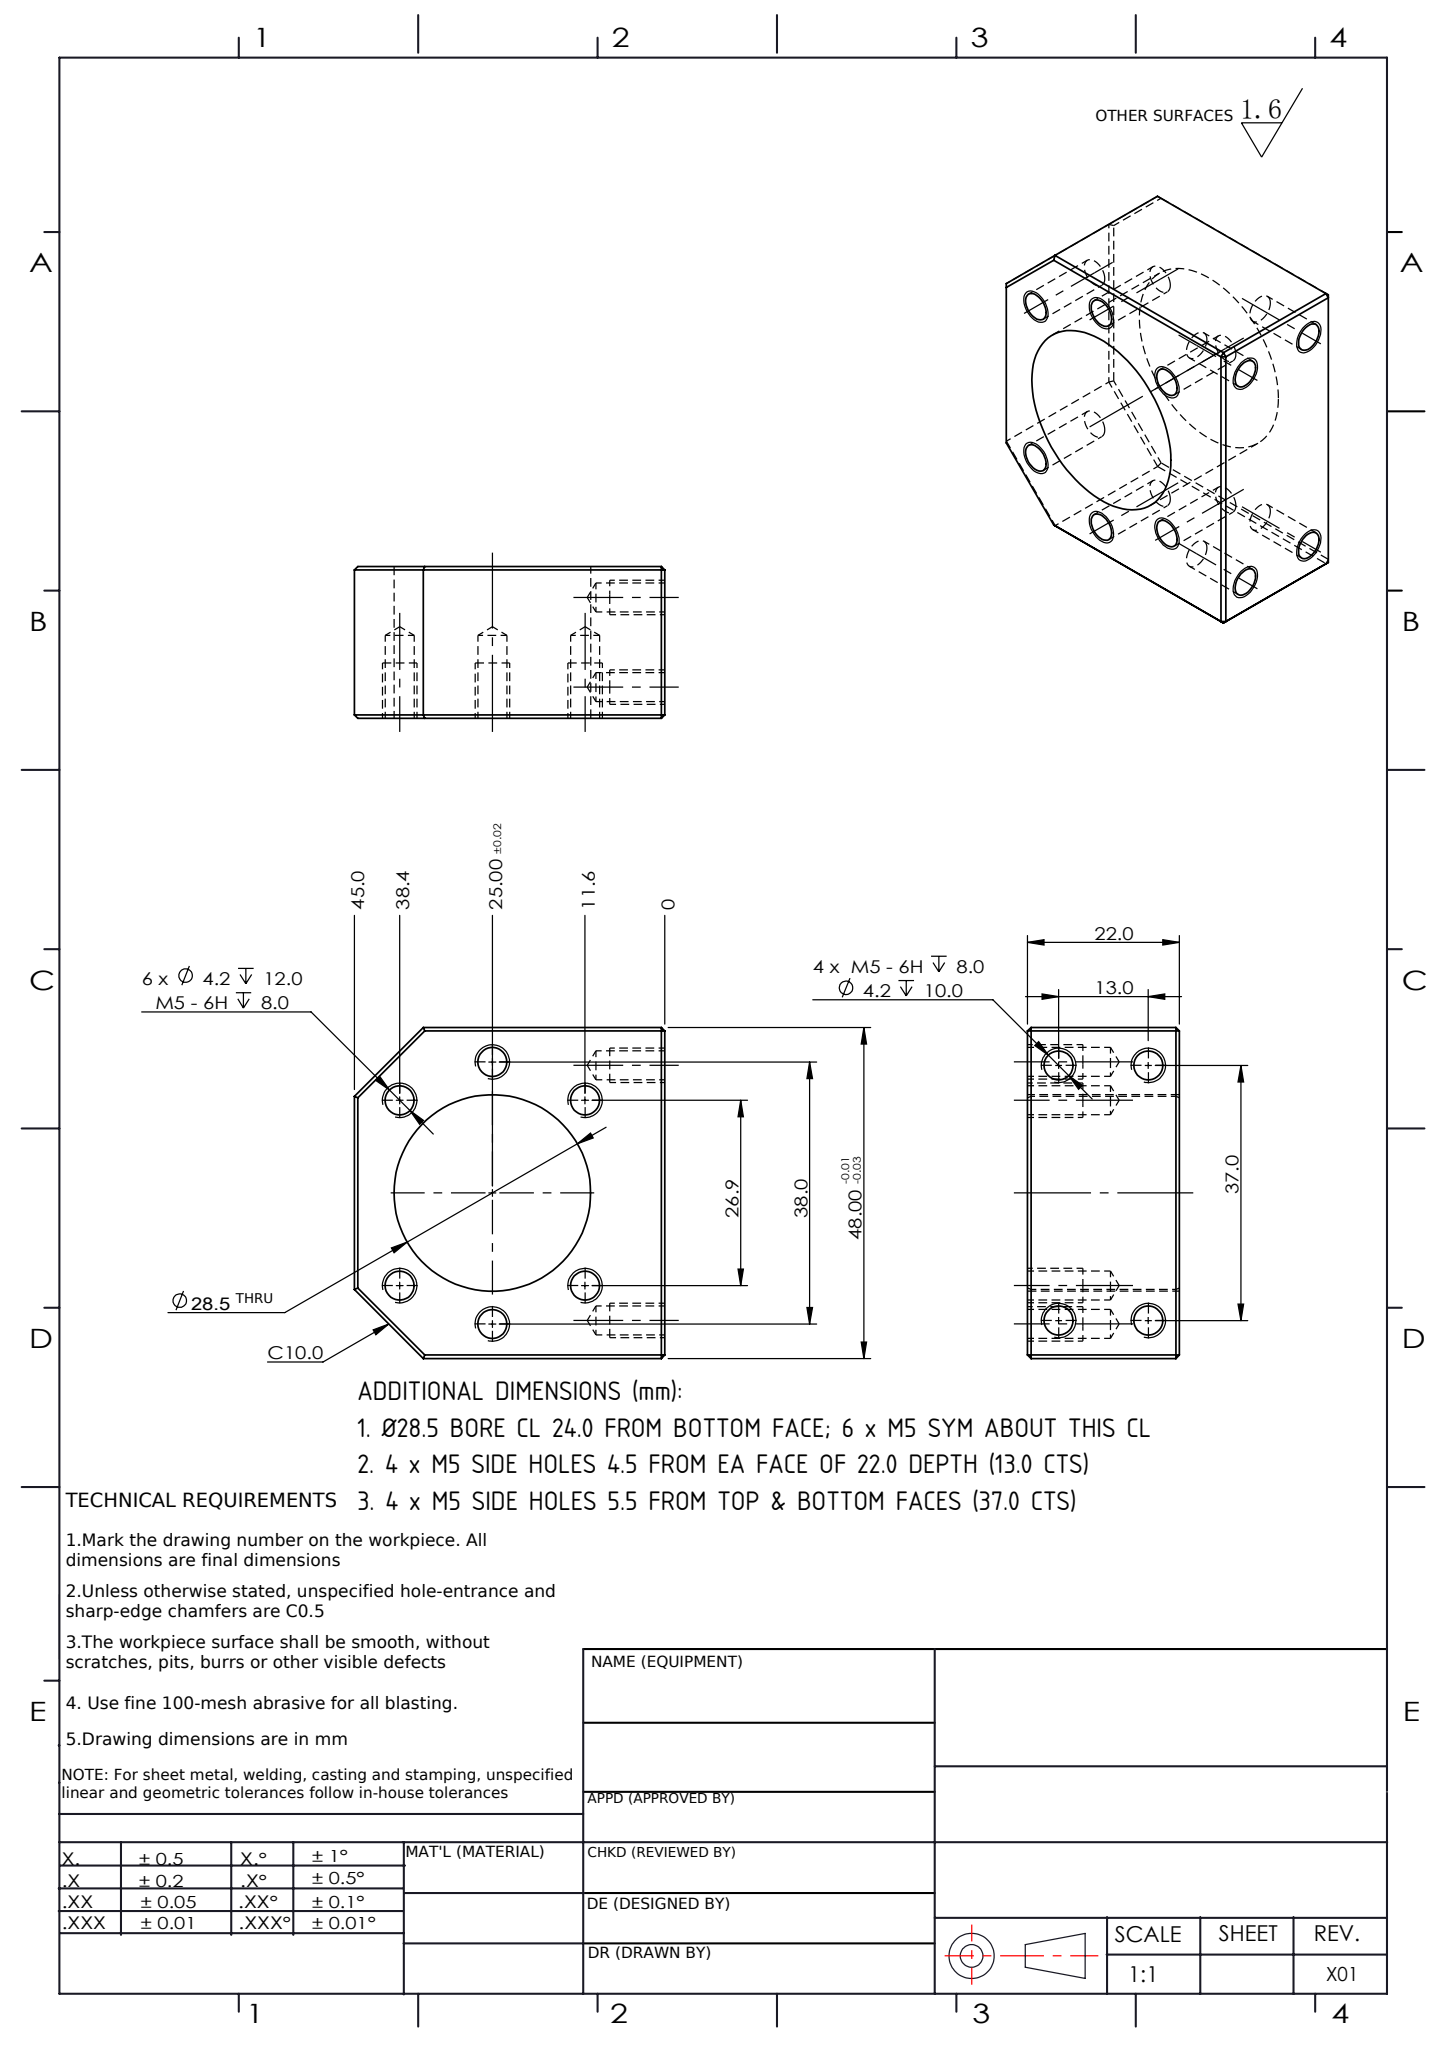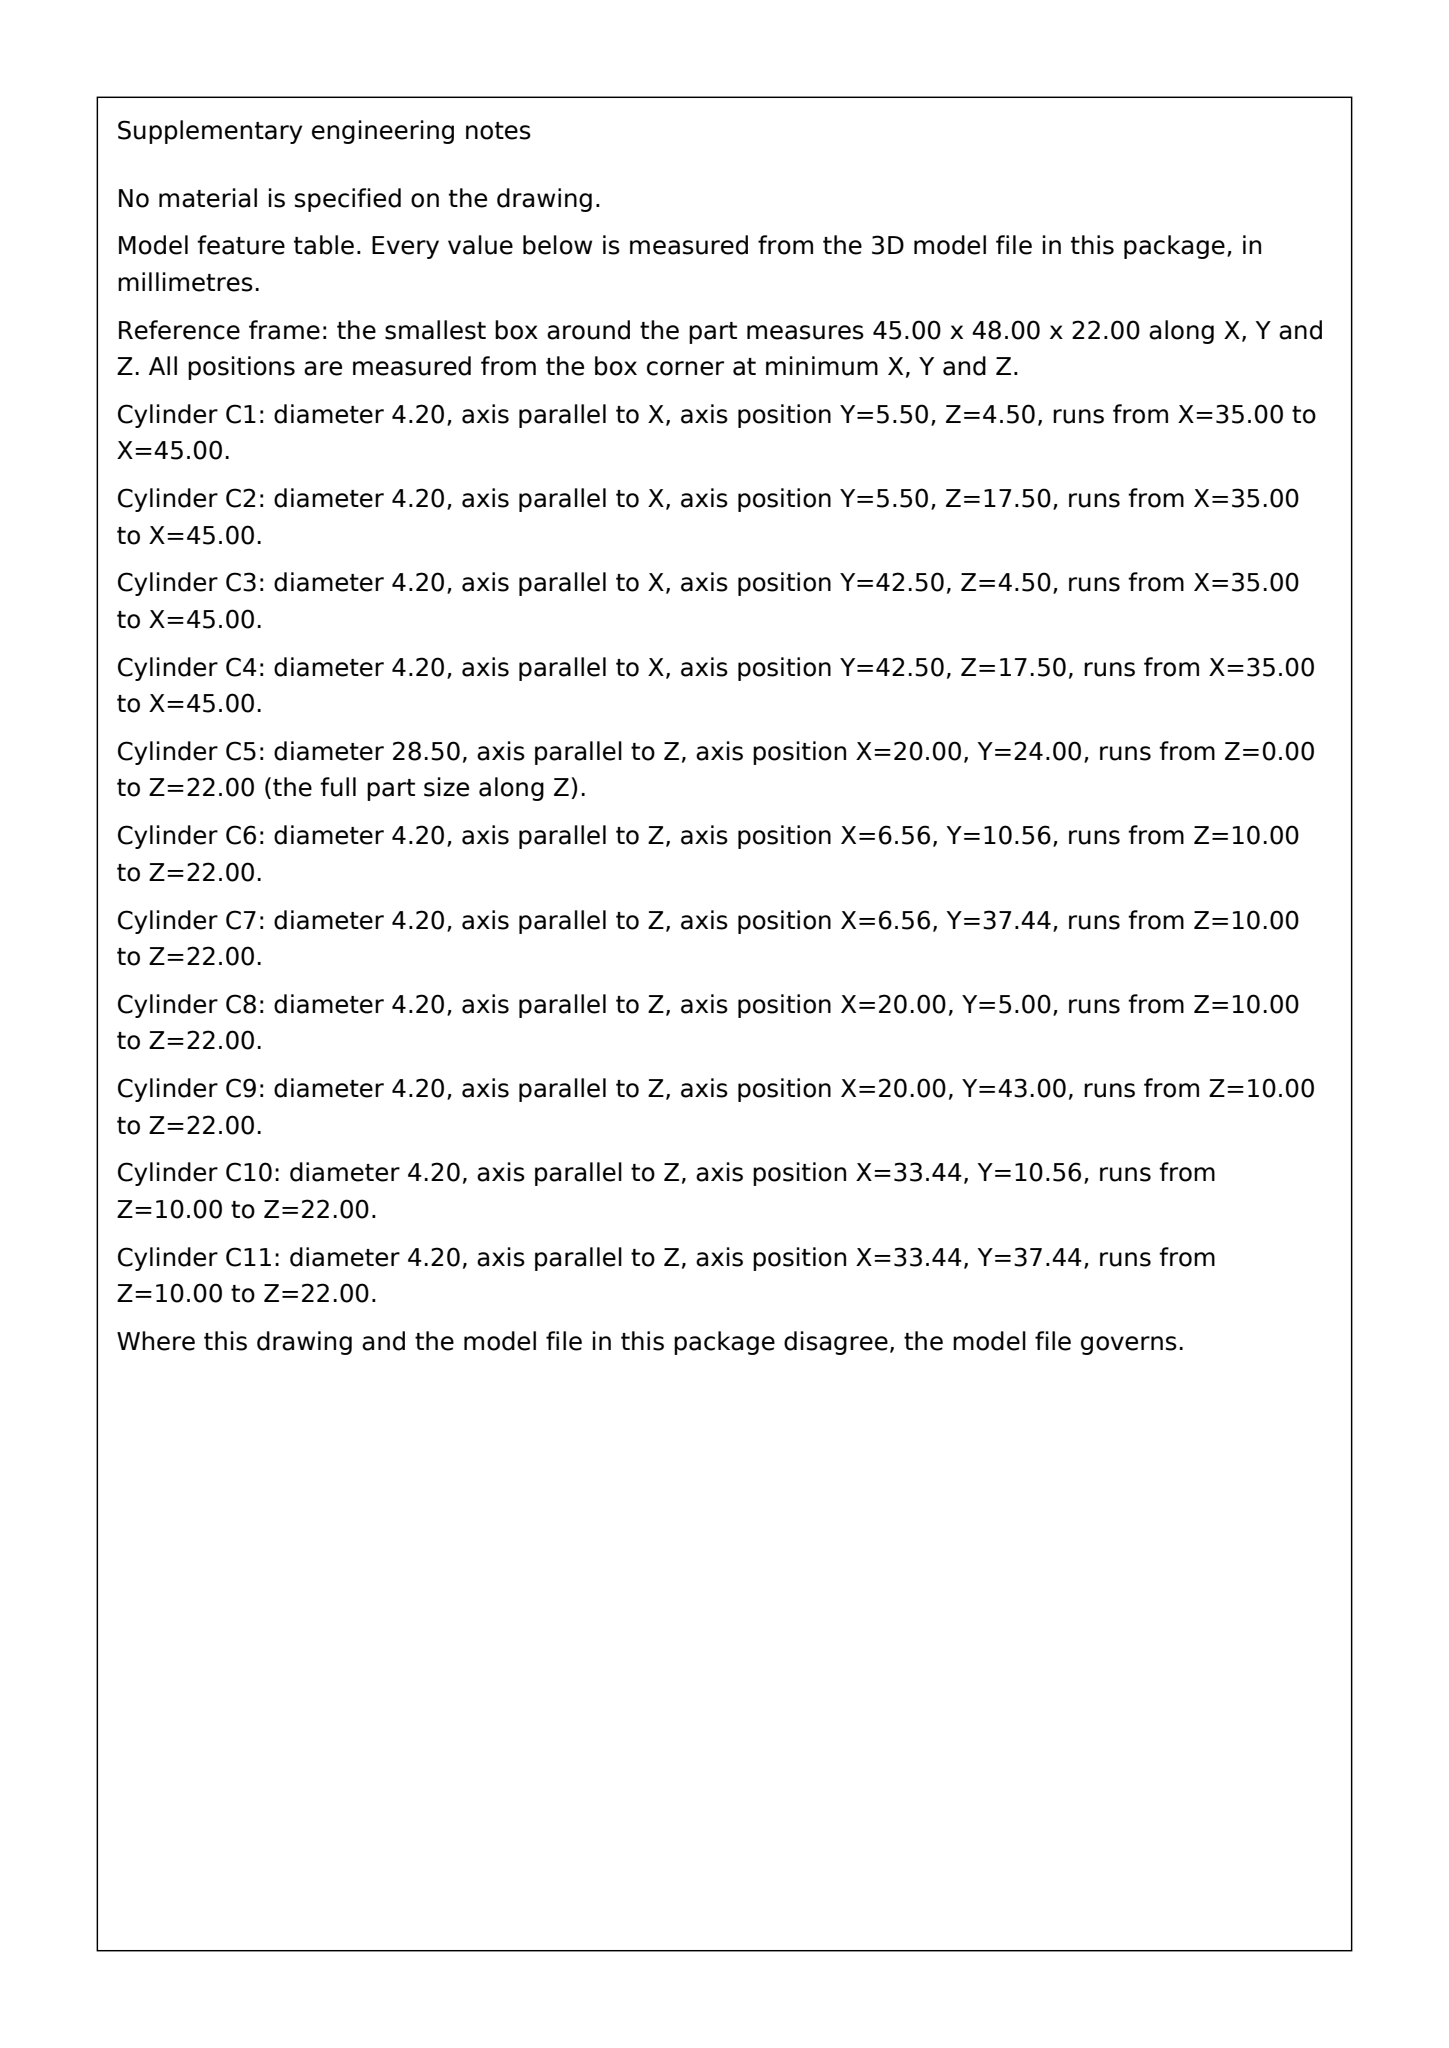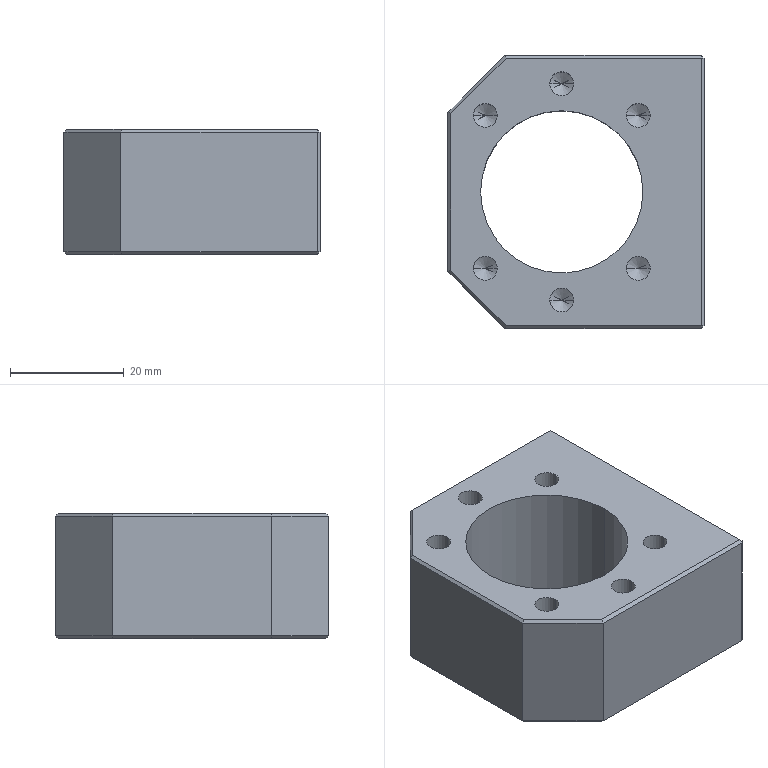Part | SolidWorks | mm | 1 solid | 68 faces | box 45 x 48 x 22 mm | volume 29627 mm3 | plane 26 | cylinder 22 | cone 20 | commonest cylinder face diameters 4.2 x20 28.5 x2
build123d program:
from build123d import *

# Parameters (mm, degrees)
SKETCH1_W             = 45
SKETCH1_H             = 48
BOSS_EXTRUDE1_DEPTH   = 22
SKETCH2_R             = 14.25
CUT_EXTRUDE1_DEPTH    = 40.576
M5_TAPPED_HOLE2_D     = 4.2
M5_TAPPED_HOLE2_DEPTH = 10
M5_TAPPED_HOLE2_TIP   = 1.262
CHAMFER1_SIZE         = 10
M5_TAPPED_HOLE3_D     = 4.2
M5_TAPPED_HOLE3_DEPTH = 12
M5_TAPPED_HOLE3_TIP   = 1.262
CHAMFER2_SIZE         = 0.5


with BuildPart() as part:
    # Sketch1 → Boss-Extrude1 (new body)
    with BuildSketch(Plane.XY):
        Rectangle(SKETCH1_W, SKETCH1_H)
    extrude(amount=BOSS_EXTRUDE1_DEPTH)

    # Sketch2 → Cut-Extrude1 (cut, through all)
    with BuildSketch(Plane.XY.offset(22)):
        with Locations((-2.5, 0)):
            Circle(SKETCH2_R)
    extrude(amount=-CUT_EXTRUDE1_DEPTH, mode=Mode.SUBTRACT)

    # M5 Tapped Hole2
    with Locations(Plane(origin=(22.5, 0, 0), x_dir=(0, 0, -1), z_dir=(1, 0, 0))):
        with Locations((-4.5, 18.5), (-4.5, -18.5), (-17.5, 18.5), (-17.5, -18.5)):
            Hole(M5_TAPPED_HOLE2_D / 2, depth=M5_TAPPED_HOLE2_DEPTH)
            with Locations((0, 0, -(M5_TAPPED_HOLE2_DEPTH + M5_TAPPED_HOLE2_TIP / 2))):  # 118° drill point
                Cone(0, M5_TAPPED_HOLE2_D / 2, M5_TAPPED_HOLE2_TIP, mode=Mode.SUBTRACT)

    # Chamfer1
    chamfer1_edges = [part.edges().sort_by_distance(p)[0] for p in [
        (-22.5, -24, 11),
        (-22.5, 24, 11),
    ]]
    chamfer(chamfer1_edges, length=CHAMFER1_SIZE)

    # M5 Tapped Hole3
    with Locations(Plane.XY.offset(22)):
        with Locations((10.935, -13.435), (-2.5, -19), (-15.935, -13.435), (-15.935, 13.435), (-2.5, 19), (10.935, 13.435)):
            Hole(M5_TAPPED_HOLE3_D / 2, depth=M5_TAPPED_HOLE3_DEPTH)
            with Locations((0, 0, -(M5_TAPPED_HOLE3_DEPTH + M5_TAPPED_HOLE3_TIP / 2))):  # 118° drill point
                Cone(0, M5_TAPPED_HOLE3_D / 2, M5_TAPPED_HOLE3_TIP, mode=Mode.SUBTRACT)

    # Chamfer2
    chamfer2_edges = [part.edges().sort_by_distance(p)[0] for p in [
        (5, -24, 0),
        (5, -24, 22),
        (-22.5, 0, 0),
        (-17.5, 19, 0),
        (-17.5, -19, 0),
        (-22.5, 0, 22),
        (22.5, 0, 22),
        (-17.5, 19, 22),
        (-17.5, -19, 22),
        (5, 24, 0),
        (22.5, 0, 0),
        (5, 24, 22),
        (22.5, -24, 11),
        (22.5, 24, 11),
    ]]
    chamfer(chamfer2_edges, length=CHAMFER2_SIZE)


solid = part.part